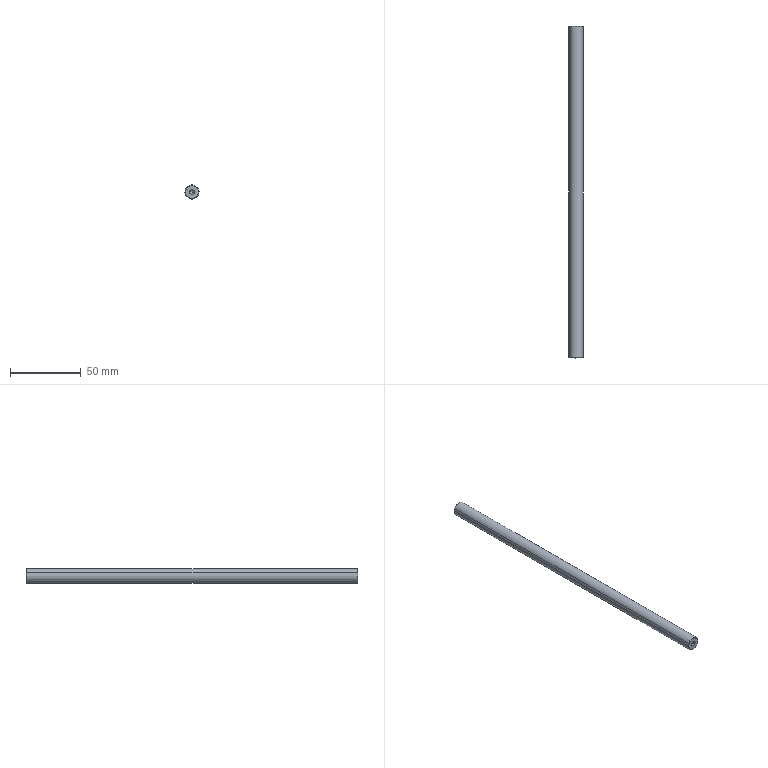Component | SolidWorks | DZ.KX.203-TC1505-30-09-01-05-07-2 | 1 solid | 16 faces | box 10 x 235 x 10 mm | volume 18211 mm3 | cone 8 | cylinder 6 | plane 2 | commonest cylinder face diameters 3.3 x4 10 x2 | material Malleable Cast Iron
build123d program:
from build123d import *

# Parameters (mm, degrees)
SKETCH1_R             = 5
BOSS_EXTRUDE1_DEPTH   = 235
M4_TAPPED_HOLE1_D     = 3.3
M4_TAPPED_HOLE1_DEPTH = 17.1
M4_TAPPED_HOLE1_TIP   = 0.9914
M4_TAPPED_HOLE2_D     = 3.3
M4_TAPPED_HOLE2_DEPTH = 10.1
M4_TAPPED_HOLE2_TIP   = 0.9914
CHAMFER2_SIZE         = 0.5


with BuildPart() as part:
    # Sketch1 → Boss-Extrude1 (new body)
    with BuildSketch(Plane(origin=(0, 0, 0), x_dir=(0, 0, -1), z_dir=(1, 0, 0))):
        with Locations(Location((0, 0, 0), (0, 0, 180))):
            Circle(SKETCH1_R)
    extrude(amount=BOSS_EXTRUDE1_DEPTH)

    # M4 Tapped Hole1
    with Locations(Plane.ZY):
        with Locations((0, 0)):
            Hole(M4_TAPPED_HOLE1_D / 2, depth=M4_TAPPED_HOLE1_DEPTH)
            with Locations((0, 0, -(M4_TAPPED_HOLE1_DEPTH + M4_TAPPED_HOLE1_TIP / 2))):  # 118° drill point
                Cone(0, M4_TAPPED_HOLE1_D / 2, M4_TAPPED_HOLE1_TIP, mode=Mode.SUBTRACT)

    # M4 Tapped Hole2
    with Locations(Plane(origin=(235, 0, 0), x_dir=(0, 0, -1), z_dir=(1, 0, 0))):
        with Locations((0, 0)):
            Hole(M4_TAPPED_HOLE2_D / 2, depth=M4_TAPPED_HOLE2_DEPTH)
            with Locations((0, 0, -(M4_TAPPED_HOLE2_DEPTH + M4_TAPPED_HOLE2_TIP / 2))):  # 118° drill point
                Cone(0, M4_TAPPED_HOLE2_D / 2, M4_TAPPED_HOLE2_TIP, mode=Mode.SUBTRACT)

    # Chamfer2
    chamfer2_edges = [part.edges().sort_by_distance(p)[0] for p in [
        (0, 0, -5),
        (235, 0, -5),
    ]]
    chamfer(chamfer2_edges, length=CHAMFER2_SIZE)


solid = part.part

# Placed as in the assembly
solid = solid.moved(Location((294.5, -796.807, -22.94), (0, 0, 90)))
STEP:
#1=COLOUR_RGB('',0.7922,0.8196,0.9333);
#2=FILL_AREA_STYLE_COLOUR('',#1);
#3=FILL_AREA_STYLE('',(#2));
#4=SURFACE_STYLE_FILL_AREA(#3);
#5=SURFACE_SIDE_STYLE('',(#4));
#6=SURFACE_STYLE_USAGE(.BOTH.,#5);
#7=PRESENTATION_STYLE_ASSIGNMENT((#6));
#8=CARTESIAN_POINT('',(11.437,-31.37,-0.8223));
#9=VERTEX_POINT('',#8);
#10=CARTESIAN_POINT('',(11.752,-31.37,-0.9841));
#11=VERTEX_POINT('',#10);
#12=CARTESIAN_POINT('',(11.594,-31.37,-0.9032));
#13=DIRECTION('',(0.,-1.,-0.));
#14=DIRECTION('',(0.8897,0.,-0.4566));
#15=AXIS2_PLACEMENT_3D('',#12,#13,#14);
#16=CIRCLE('',#15,0.1772);
#17=EDGE_CURVE('',#9,#11,#16,.T.);
#18=ORIENTED_EDGE('',*,*,#17,.F.);
#19=CARTESIAN_POINT('',(11.419,-31.351,-0.8133));
#20=VERTEX_POINT('',#19);
#21=CARTESIAN_POINT('',(11.419,-31.351,-0.8133));
#22=DIRECTION('',(-0.6291,0.7071,0.3228));
#23=VECTOR('',#22,39.37);
#24=LINE('',#21,#23);
#25=EDGE_CURVE('',#9,#20,#24,.T.);
#26=ORIENTED_EDGE('',*,*,#25,.T.);
#27=CARTESIAN_POINT('',(11.77,-31.351,-0.993));
#28=VERTEX_POINT('',#27);
#29=CARTESIAN_POINT('',(11.594,-31.351,-0.9032));
#30=DIRECTION('',(-0.,1.,0.));
#31=DIRECTION('',(0.8897,0.,-0.4566));
#32=AXIS2_PLACEMENT_3D('',#29,#30,#31);
#33=CIRCLE('',#32,0.1969);
#34=EDGE_CURVE('',#28,#20,#33,.T.);
#35=ORIENTED_EDGE('',*,*,#34,.F.);
#36=CARTESIAN_POINT('',(11.77,-31.351,-0.993));
#37=DIRECTION('',(0.6291,0.7071,-0.3228));
#38=VECTOR('',#37,39.37);
#39=LINE('',#36,#38);
#40=EDGE_CURVE('',#11,#28,#39,.T.);
#41=ORIENTED_EDGE('',*,*,#40,.F.);
#42=EDGE_LOOP('',(#18,#26,#35,#41));
#43=FACE_OUTER_BOUND('',#42,.T.);
#44=CARTESIAN_POINT('',(11.594,-31.351,-0.9032));
#45=DIRECTION('',(-0.,1.,0.));
#46=DIRECTION('',(0.8897,0.,-0.4566));
#47=AXIS2_PLACEMENT_3D('',#44,#45,#46);
#48=CONICAL_SURFACE('',#47,0.1969,0.7854);
#49=ADVANCED_FACE('',(#43),#48,.T.);
#50=CARTESIAN_POINT('',(11.752,-22.118,-0.9841));
#51=VERTEX_POINT('',#50);
#52=CARTESIAN_POINT('',(11.437,-22.118,-0.8223));
#53=VERTEX_POINT('',#52);
#54=CARTESIAN_POINT('',(11.594,-22.118,-0.9032));
#55=DIRECTION('',(-0.,1.,0.));
#56=DIRECTION('',(0.8897,0.,-0.4566));
#57=AXIS2_PLACEMENT_3D('',#54,#55,#56);
#58=CIRCLE('',#57,0.1772);
#59=EDGE_CURVE('',#51,#53,#58,.T.);
#60=ORIENTED_EDGE('',*,*,#59,.F.);
#61=CARTESIAN_POINT('',(11.77,-22.138,-0.993));
#62=VERTEX_POINT('',#61);
#63=CARTESIAN_POINT('',(11.752,-22.118,-0.9841));
#64=DIRECTION('',(0.6291,-0.7071,-0.3228));
#65=VECTOR('',#64,39.37);
#66=LINE('',#63,#65);
#67=EDGE_CURVE('',#51,#62,#66,.T.);
#68=ORIENTED_EDGE('',*,*,#67,.T.);
#69=CARTESIAN_POINT('',(11.419,-22.138,-0.8133));
#70=VERTEX_POINT('',#69);
#71=CARTESIAN_POINT('',(11.594,-22.138,-0.9032));
#72=DIRECTION('',(0.,-1.,-0.));
#73=DIRECTION('',(0.8897,0.,-0.4566));
#74=AXIS2_PLACEMENT_3D('',#71,#72,#73);
#75=CIRCLE('',#74,0.1969);
#76=EDGE_CURVE('',#70,#62,#75,.T.);
#77=ORIENTED_EDGE('',*,*,#76,.F.);
#78=CARTESIAN_POINT('',(11.437,-22.118,-0.8223));
#79=DIRECTION('',(-0.6291,-0.7071,0.3228));
#80=VECTOR('',#79,39.37);
#81=LINE('',#78,#80);
#82=EDGE_CURVE('',#53,#70,#81,.T.);
#83=ORIENTED_EDGE('',*,*,#82,.F.);
#84=EDGE_LOOP('',(#60,#68,#77,#83));
#85=FACE_OUTER_BOUND('',#84,.T.);
#86=CARTESIAN_POINT('',(11.594,-22.118,-0.9032));
#87=DIRECTION('',(0.,-1.,-0.));
#88=DIRECTION('',(-0.8897,0.,0.4566));
#89=AXIS2_PLACEMENT_3D('',#86,#87,#88);
#90=CONICAL_SURFACE('',#89,0.1772,0.7854);
#91=ADVANCED_FACE('',(#85),#90,.T.);
#92=CARTESIAN_POINT('',(11.537,-22.516,-0.8735));
#93=VERTEX_POINT('',#92);
#94=CARTESIAN_POINT('',(11.652,-22.516,-0.9328));
#95=VERTEX_POINT('',#94);
#96=CARTESIAN_POINT('',(11.594,-22.516,-0.9032));
#97=DIRECTION('',(-0.,1.,0.));
#98=DIRECTION('',(0.8897,0.,-0.4566));
#99=AXIS2_PLACEMENT_3D('',#96,#97,#98);
#100=CIRCLE('',#99,0.06496);
#101=EDGE_CURVE('',#93,#95,#100,.T.);
#102=ORIENTED_EDGE('',*,*,#101,.F.);
#103=CARTESIAN_POINT('',(11.537,-22.118,-0.8735));
#104=VERTEX_POINT('',#103);
#105=CARTESIAN_POINT('',(11.537,-22.118,-0.8735));
#106=DIRECTION('',(-0.,1.,0.));
#107=VECTOR('',#106,39.37);
#108=LINE('',#105,#107);
#109=EDGE_CURVE('',#93,#104,#108,.T.);
#110=ORIENTED_EDGE('',*,*,#109,.T.);
#111=CARTESIAN_POINT('',(11.652,-22.118,-0.9328));
#112=VERTEX_POINT('',#111);
#113=CARTESIAN_POINT('',(11.594,-22.118,-0.9032));
#114=DIRECTION('',(-0.,1.,0.));
#115=DIRECTION('',(0.8897,0.,-0.4566));
#116=AXIS2_PLACEMENT_3D('',#113,#114,#115);
#117=CIRCLE('',#116,0.06496);
#118=EDGE_CURVE('',#104,#112,#117,.T.);
#119=ORIENTED_EDGE('',*,*,#118,.T.);
#120=CARTESIAN_POINT('',(11.652,-22.118,-0.9328));
#121=DIRECTION('',(-0.,1.,0.));
#122=VECTOR('',#121,39.37);
#123=LINE('',#120,#122);
#124=EDGE_CURVE('',#95,#112,#123,.T.);
#125=ORIENTED_EDGE('',*,*,#124,.F.);
#126=EDGE_LOOP('',(#102,#110,#119,#125));
#127=FACE_OUTER_BOUND('',#126,.T.);
#128=CARTESIAN_POINT('',(11.594,-22.118,-0.9032));
#129=DIRECTION('',(-0.,1.,0.));
#130=DIRECTION('',(0.8897,0.,-0.4566));
#131=AXIS2_PLACEMENT_3D('',#128,#129,#130);
#132=CYLINDRICAL_SURFACE('',#131,0.06496);
#133=ADVANCED_FACE('',(#127),#132,.F.);
#134=CARTESIAN_POINT('',(11.594,-22.555,-0.9032));
#135=VERTEX_POINT('',#134);
#136=CARTESIAN_POINT('',(11.652,-22.516,-0.9328));
#137=DIRECTION('',(0.7626,0.515,-0.3914));
#138=VECTOR('',#137,39.37);
#139=LINE('',#136,#138);
#140=EDGE_CURVE('',#135,#95,#139,.T.);
#141=ORIENTED_EDGE('',*,*,#140,.F.);
#142=CARTESIAN_POINT('',(11.537,-22.516,-0.8735));
#143=DIRECTION('',(-0.7626,0.515,0.3914));
#144=VECTOR('',#143,39.37);
#145=LINE('',#142,#144);
#146=EDGE_CURVE('',#135,#93,#145,.T.);
#147=ORIENTED_EDGE('',*,*,#146,.T.);
#148=ORIENTED_EDGE('',*,*,#101,.T.);
#149=EDGE_LOOP('',(#141,#147,#148));
#150=FACE_OUTER_BOUND('',#149,.T.);
#151=CARTESIAN_POINT('',(11.594,-22.516,-0.9032));
#152=DIRECTION('',(-0.,1.,0.));
#153=DIRECTION('',(0.8897,0.,-0.4566));
#154=AXIS2_PLACEMENT_3D('',#151,#152,#153);
#155=CONICAL_SURFACE('',#154,0.06496,1.03);
#156=ADVANCED_FACE('',(#150),#155,.F.);
#157=CARTESIAN_POINT('',(11.652,-30.697,-0.9328));
#158=VERTEX_POINT('',#157);
#159=CARTESIAN_POINT('',(11.537,-30.697,-0.8735));
#160=VERTEX_POINT('',#159);
#161=CARTESIAN_POINT('',(11.594,-30.697,-0.9032));
#162=DIRECTION('',(0.,-1.,-0.));
#163=DIRECTION('',(-0.8897,0.,0.4566));
#164=AXIS2_PLACEMENT_3D('',#161,#162,#163);
#165=CIRCLE('',#164,0.06496);
#166=EDGE_CURVE('',#158,#160,#165,.T.);
#167=ORIENTED_EDGE('',*,*,#166,.F.);
#168=CARTESIAN_POINT('',(11.652,-31.37,-0.9328));
#169=VERTEX_POINT('',#168);
#170=CARTESIAN_POINT('',(11.652,-31.37,-0.9328));
#171=DIRECTION('',(0.,-1.,-0.));
#172=VECTOR('',#171,39.37);
#173=LINE('',#170,#172);
#174=EDGE_CURVE('',#158,#169,#173,.T.);
#175=ORIENTED_EDGE('',*,*,#174,.T.);
#176=CARTESIAN_POINT('',(11.537,-31.37,-0.8735));
#177=VERTEX_POINT('',#176);
#178=CARTESIAN_POINT('',(11.594,-31.37,-0.9032));
#179=DIRECTION('',(0.,-1.,-0.));
#180=DIRECTION('',(-0.8897,0.,0.4566));
#181=AXIS2_PLACEMENT_3D('',#178,#179,#180);
#182=CIRCLE('',#181,0.06496);
#183=EDGE_CURVE('',#169,#177,#182,.T.);
#184=ORIENTED_EDGE('',*,*,#183,.T.);
#185=CARTESIAN_POINT('',(11.537,-31.37,-0.8735));
#186=DIRECTION('',(0.,-1.,-0.));
#187=VECTOR('',#186,39.37);
#188=LINE('',#185,#187);
#189=EDGE_CURVE('',#160,#177,#188,.T.);
#190=ORIENTED_EDGE('',*,*,#189,.F.);
#191=EDGE_LOOP('',(#167,#175,#184,#190));
#192=FACE_OUTER_BOUND('',#191,.T.);
#193=CARTESIAN_POINT('',(11.594,-31.37,-0.9032));
#194=DIRECTION('',(0.,-1.,-0.));
#195=DIRECTION('',(-0.8897,0.,0.4566));
#196=AXIS2_PLACEMENT_3D('',#193,#194,#195);
#197=CYLINDRICAL_SURFACE('',#196,0.06496);
#198=ADVANCED_FACE('',(#192),#197,.F.);
#199=CARTESIAN_POINT('',(11.594,-30.658,-0.9032));
#200=VERTEX_POINT('',#199);
#201=CARTESIAN_POINT('',(11.537,-30.697,-0.8735));
#202=DIRECTION('',(-0.7626,-0.515,0.3914));
#203=VECTOR('',#202,39.37);
#204=LINE('',#201,#203);
#205=EDGE_CURVE('',#200,#160,#204,.T.);
#206=ORIENTED_EDGE('',*,*,#205,.F.);
#207=CARTESIAN_POINT('',(11.652,-30.697,-0.9328));
#208=DIRECTION('',(0.7626,-0.515,-0.3914));
#209=VECTOR('',#208,39.37);
#210=LINE('',#207,#209);
#211=EDGE_CURVE('',#200,#158,#210,.T.);
#212=ORIENTED_EDGE('',*,*,#211,.T.);
#213=ORIENTED_EDGE('',*,*,#166,.T.);
#214=EDGE_LOOP('',(#206,#212,#213));
#215=FACE_OUTER_BOUND('',#214,.T.);
#216=CARTESIAN_POINT('',(11.594,-30.697,-0.9032));
#217=DIRECTION('',(0.,-1.,-0.));
#218=DIRECTION('',(-0.8897,0.,0.4566));
#219=AXIS2_PLACEMENT_3D('',#216,#217,#218);
#220=CONICAL_SURFACE('',#219,0.06496,1.03);
#221=ADVANCED_FACE('',(#215),#220,.F.);
#222=ORIENTED_EDGE('',*,*,#76,.T.);
#223=CARTESIAN_POINT('',(11.77,-22.118,-0.993));
#224=DIRECTION('',(0.,-1.,-0.));
#225=VECTOR('',#224,39.37);
#226=LINE('',#223,#225);
#227=EDGE_CURVE('',#62,#28,#226,.T.);
#228=ORIENTED_EDGE('',*,*,#227,.T.);
#229=ORIENTED_EDGE('',*,*,#34,.T.);
#230=CARTESIAN_POINT('',(11.419,-22.118,-0.8133));
#231=DIRECTION('',(0.,-1.,-0.));
#232=VECTOR('',#231,39.37);
#233=LINE('',#230,#232);
#234=EDGE_CURVE('',#70,#20,#233,.T.);
#235=ORIENTED_EDGE('',*,*,#234,.F.);
#236=EDGE_LOOP('',(#222,#228,#229,#235));
#237=FACE_OUTER_BOUND('',#236,.T.);
#238=CARTESIAN_POINT('',(11.594,-22.118,-0.9032));
#239=DIRECTION('',(0.,-1.,-0.));
#240=DIRECTION('',(-0.8897,0.,0.4566));
#241=AXIS2_PLACEMENT_3D('',#238,#239,#240);
#242=CYLINDRICAL_SURFACE('',#241,0.1969);
#243=ADVANCED_FACE('',(#237),#242,.T.);
#244=ORIENTED_EDGE('',*,*,#227,.F.);
#245=CARTESIAN_POINT('',(11.594,-22.138,-0.9032));
#246=DIRECTION('',(0.,-1.,-0.));
#247=DIRECTION('',(0.8897,0.,-0.4566));
#248=AXIS2_PLACEMENT_3D('',#245,#246,#247);
#249=CIRCLE('',#248,0.1969);
#250=EDGE_CURVE('',#62,#70,#249,.T.);
#251=ORIENTED_EDGE('',*,*,#250,.T.);
#252=ORIENTED_EDGE('',*,*,#234,.T.);
#253=CARTESIAN_POINT('',(11.594,-31.351,-0.9032));
#254=DIRECTION('',(-0.,1.,0.));
#255=DIRECTION('',(0.8897,0.,-0.4566));
#256=AXIS2_PLACEMENT_3D('',#253,#254,#255);
#257=CIRCLE('',#256,0.1969);
#258=EDGE_CURVE('',#20,#28,#257,.T.);
#259=ORIENTED_EDGE('',*,*,#258,.T.);
#260=EDGE_LOOP('',(#244,#251,#252,#259));
#261=FACE_OUTER_BOUND('',#260,.T.);
#262=CARTESIAN_POINT('',(11.594,-22.118,-0.9032));
#263=DIRECTION('',(0.,-1.,-0.));
#264=DIRECTION('',(-0.8897,0.,0.4566));
#265=AXIS2_PLACEMENT_3D('',#262,#263,#264);
#266=CYLINDRICAL_SURFACE('',#265,0.1969);
#267=ADVANCED_FACE('',(#261),#266,.T.);
#268=CARTESIAN_POINT('',(11.594,-22.118,-0.9032));
#269=DIRECTION('',(-0.,1.,0.));
#270=DIRECTION('',(0.8897,0.,-0.4566));
#271=AXIS2_PLACEMENT_3D('',#268,#269,#270);
#272=CIRCLE('',#271,0.1772);
#273=EDGE_CURVE('',#53,#51,#272,.T.);
#274=ORIENTED_EDGE('',*,*,#273,.T.);
#275=ORIENTED_EDGE('',*,*,#59,.T.);
#276=EDGE_LOOP('',(#274,#275));
#277=FACE_OUTER_BOUND('',#276,.T.);
#278=CARTESIAN_POINT('',(11.594,-22.118,-0.9032));
#279=DIRECTION('',(-0.,1.,0.));
#280=DIRECTION('',(0.8897,0.,-0.4566));
#281=AXIS2_PLACEMENT_3D('',#278,#279,#280);
#282=CIRCLE('',#281,0.06496);
#283=EDGE_CURVE('',#112,#104,#282,.T.);
#284=ORIENTED_EDGE('',*,*,#283,.F.);
#285=ORIENTED_EDGE('',*,*,#118,.F.);
#286=EDGE_LOOP('',(#284,#285));
#287=FACE_BOUND('',#286,.T.);
#288=CARTESIAN_POINT('',(11.594,-22.118,-0.9032));
#289=DIRECTION('',(-0.,1.,0.));
#290=DIRECTION('',(0.8897,0.,-0.4566));
#291=AXIS2_PLACEMENT_3D('',#288,#289,#290);
#292=PLANE('',#291);
#293=ADVANCED_FACE('',(#277,#287),#292,.T.);
#294=CARTESIAN_POINT('',(11.594,-31.37,-0.9032));
#295=DIRECTION('',(0.,-1.,-0.));
#296=DIRECTION('',(0.8897,0.,-0.4566));
#297=AXIS2_PLACEMENT_3D('',#294,#295,#296);
#298=CIRCLE('',#297,0.1772);
#299=EDGE_CURVE('',#11,#9,#298,.T.);
#300=ORIENTED_EDGE('',*,*,#299,.T.);
#301=ORIENTED_EDGE('',*,*,#17,.T.);
#302=EDGE_LOOP('',(#300,#301));
#303=FACE_OUTER_BOUND('',#302,.T.);
#304=CARTESIAN_POINT('',(11.594,-31.37,-0.9032));
#305=DIRECTION('',(0.,-1.,-0.));
#306=DIRECTION('',(-0.8897,0.,0.4566));
#307=AXIS2_PLACEMENT_3D('',#304,#305,#306);
#308=CIRCLE('',#307,0.06496);
#309=EDGE_CURVE('',#177,#169,#308,.T.);
#310=ORIENTED_EDGE('',*,*,#309,.F.);
#311=ORIENTED_EDGE('',*,*,#183,.F.);
#312=EDGE_LOOP('',(#310,#311));
#313=FACE_BOUND('',#312,.T.);
#314=CARTESIAN_POINT('',(11.594,-31.37,-0.9032));
#315=DIRECTION('',(-0.,1.,0.));
#316=DIRECTION('',(0.8897,0.,-0.4566));
#317=AXIS2_PLACEMENT_3D('',#314,#315,#316);
#318=PLANE('',#317);
#319=ADVANCED_FACE('',(#303,#313),#318,.F.);
#320=ORIENTED_EDGE('',*,*,#211,.F.);
#321=ORIENTED_EDGE('',*,*,#205,.T.);
#322=CARTESIAN_POINT('',(11.594,-30.697,-0.9032));
#323=DIRECTION('',(0.,-1.,-0.));
#324=DIRECTION('',(-0.8897,0.,0.4566));
#325=AXIS2_PLACEMENT_3D('',#322,#323,#324);
#326=CIRCLE('',#325,0.06496);
#327=EDGE_CURVE('',#160,#158,#326,.T.);
#328=ORIENTED_EDGE('',*,*,#327,.T.);
#329=EDGE_LOOP('',(#320,#321,#328));
#330=FACE_OUTER_BOUND('',#329,.T.);
#331=CARTESIAN_POINT('',(11.594,-30.697,-0.9032));
#332=DIRECTION('',(0.,-1.,-0.));
#333=DIRECTION('',(-0.8897,0.,0.4566));
#334=AXIS2_PLACEMENT_3D('',#331,#332,#333);
#335=CONICAL_SURFACE('',#334,0.06496,1.03);
#336=ADVANCED_FACE('',(#330),#335,.F.);
#337=ORIENTED_EDGE('',*,*,#174,.F.);
#338=ORIENTED_EDGE('',*,*,#327,.F.);
#339=ORIENTED_EDGE('',*,*,#189,.T.);
#340=ORIENTED_EDGE('',*,*,#309,.T.);
#341=EDGE_LOOP('',(#337,#338,#339,#340));
#342=FACE_OUTER_BOUND('',#341,.T.);
#343=CARTESIAN_POINT('',(11.594,-31.37,-0.9032));
#344=DIRECTION('',(0.,-1.,-0.));
#345=DIRECTION('',(-0.8897,0.,0.4566));
#346=AXIS2_PLACEMENT_3D('',#343,#344,#345);
#347=CYLINDRICAL_SURFACE('',#346,0.06496);
#348=ADVANCED_FACE('',(#342),#347,.F.);
#349=ORIENTED_EDGE('',*,*,#146,.F.);
#350=ORIENTED_EDGE('',*,*,#140,.T.);
#351=CARTESIAN_POINT('',(11.594,-22.516,-0.9032));
#352=DIRECTION('',(-0.,1.,0.));
#353=DIRECTION('',(0.8897,0.,-0.4566));
#354=AXIS2_PLACEMENT_3D('',#351,#352,#353);
#355=CIRCLE('',#354,0.06496);
#356=EDGE_CURVE('',#95,#93,#355,.T.);
#357=ORIENTED_EDGE('',*,*,#356,.T.);
#358=EDGE_LOOP('',(#349,#350,#357));
#359=FACE_OUTER_BOUND('',#358,.T.);
#360=CARTESIAN_POINT('',(11.594,-22.516,-0.9032));
#361=DIRECTION('',(-0.,1.,0.));
#362=DIRECTION('',(0.8897,0.,-0.4566));
#363=AXIS2_PLACEMENT_3D('',#360,#361,#362);
#364=CONICAL_SURFACE('',#363,0.06496,1.03);
#365=ADVANCED_FACE('',(#359),#364,.F.);
#366=ORIENTED_EDGE('',*,*,#109,.F.);
#367=ORIENTED_EDGE('',*,*,#356,.F.);
#368=ORIENTED_EDGE('',*,*,#124,.T.);
#369=ORIENTED_EDGE('',*,*,#283,.T.);
#370=EDGE_LOOP('',(#366,#367,#368,#369));
#371=FACE_OUTER_BOUND('',#370,.T.);
#372=CARTESIAN_POINT('',(11.594,-22.118,-0.9032));
#373=DIRECTION('',(-0.,1.,0.));
#374=DIRECTION('',(0.8897,0.,-0.4566));
#375=AXIS2_PLACEMENT_3D('',#372,#373,#374);
#376=CYLINDRICAL_SURFACE('',#375,0.06496);
#377=ADVANCED_FACE('',(#371),#376,.F.);
#378=ORIENTED_EDGE('',*,*,#67,.F.);
#379=ORIENTED_EDGE('',*,*,#273,.F.);
#380=ORIENTED_EDGE('',*,*,#82,.T.);
#381=ORIENTED_EDGE('',*,*,#250,.F.);
#382=EDGE_LOOP('',(#378,#379,#380,#381));
#383=FACE_OUTER_BOUND('',#382,.T.);
#384=CARTESIAN_POINT('',(11.594,-22.118,-0.9032));
#385=DIRECTION('',(0.,-1.,-0.));
#386=DIRECTION('',(-0.8897,0.,0.4566));
#387=AXIS2_PLACEMENT_3D('',#384,#385,#386);
#388=CONICAL_SURFACE('',#387,0.1772,0.7854);
#389=ADVANCED_FACE('',(#383),#388,.T.);
#390=ORIENTED_EDGE('',*,*,#25,.F.);
#391=ORIENTED_EDGE('',*,*,#299,.F.);
#392=ORIENTED_EDGE('',*,*,#40,.T.);
#393=ORIENTED_EDGE('',*,*,#258,.F.);
#394=EDGE_LOOP('',(#390,#391,#392,#393));
#395=FACE_OUTER_BOUND('',#394,.T.);
#396=CARTESIAN_POINT('',(11.594,-31.351,-0.9032));
#397=DIRECTION('',(-0.,1.,0.));
#398=DIRECTION('',(0.8897,0.,-0.4566));
#399=AXIS2_PLACEMENT_3D('',#396,#397,#398);
#400=CONICAL_SURFACE('',#399,0.1969,0.7854);
#401=ADVANCED_FACE('',(#395),#400,.T.);
#402=CLOSED_SHELL('',(#49,#91,#133,#156,#198,#221,#243,#267,#293,#319,#336,#348,#365,#377,#389,#401));
#403=MANIFOLD_SOLID_BREP('',#402);
#404=STYLED_ITEM('',(#7),#403);
#405=PRESENTATION_LAYER_ASSIGNMENT('','',(#404));
#406=(LENGTH_UNIT()NAMED_UNIT(*)SI_UNIT($,.METRE.));
#407=LENGTH_MEASURE_WITH_UNIT(LENGTH_MEASURE(0.0254),#406);
#408=DIMENSIONAL_EXPONENTS(1.,0.,0.,0.,0.,0.,0.);
#409=(CONVERSION_BASED_UNIT('',#407)LENGTH_UNIT()NAMED_UNIT(#408));
#410=UNCERTAINTY_MEASURE_WITH_UNIT(LENGTH_MEASURE(0.00001),#409,'','');
#411=(NAMED_UNIT(*)PLANE_ANGLE_UNIT()SI_UNIT($,.RADIAN.));
#412=(NAMED_UNIT(*)SI_UNIT($,.STERADIAN.)SOLID_ANGLE_UNIT());
#413=(GEOMETRIC_REPRESENTATION_CONTEXT(3)GLOBAL_UNCERTAINTY_ASSIGNED_CONTEXT((#410))GLOBAL_UNIT_ASSIGNED_CONTEXT((#409,#411,#412))REPRESENTATION_CONTEXT('',''));
#414=MECHANICAL_DESIGN_GEOMETRIC_PRESENTATION_REPRESENTATION('',(#404),#413);
#415=CARTESIAN_POINT('',(0.,0.,0.));
#416=DIRECTION('',(0.,0.,1.));
#417=DIRECTION('',(1.,0.,0.));
#418=AXIS2_PLACEMENT_3D('',#415,#416,#417);
#419=(LENGTH_UNIT()NAMED_UNIT(*)SI_UNIT($,.METRE.));
#420=LENGTH_MEASURE_WITH_UNIT(LENGTH_MEASURE(0.0254),#419);
#421=DIMENSIONAL_EXPONENTS(1.,0.,0.,0.,0.,0.,0.);
#422=(CONVERSION_BASED_UNIT('',#420)LENGTH_UNIT()NAMED_UNIT(#421));
#423=UNCERTAINTY_MEASURE_WITH_UNIT(LENGTH_MEASURE(0.00001),#422,'','');
#424=(NAMED_UNIT(*)PLANE_ANGLE_UNIT()SI_UNIT($,.RADIAN.));
#425=(NAMED_UNIT(*)SI_UNIT($,.STERADIAN.)SOLID_ANGLE_UNIT());
#426=(GEOMETRIC_REPRESENTATION_CONTEXT(3)GLOBAL_UNCERTAINTY_ASSIGNED_CONTEXT((#423))GLOBAL_UNIT_ASSIGNED_CONTEXT((#422,#424,#425))REPRESENTATION_CONTEXT('',''));
#427=ADVANCED_BREP_SHAPE_REPRESENTATION('',(#403,#418),#426);